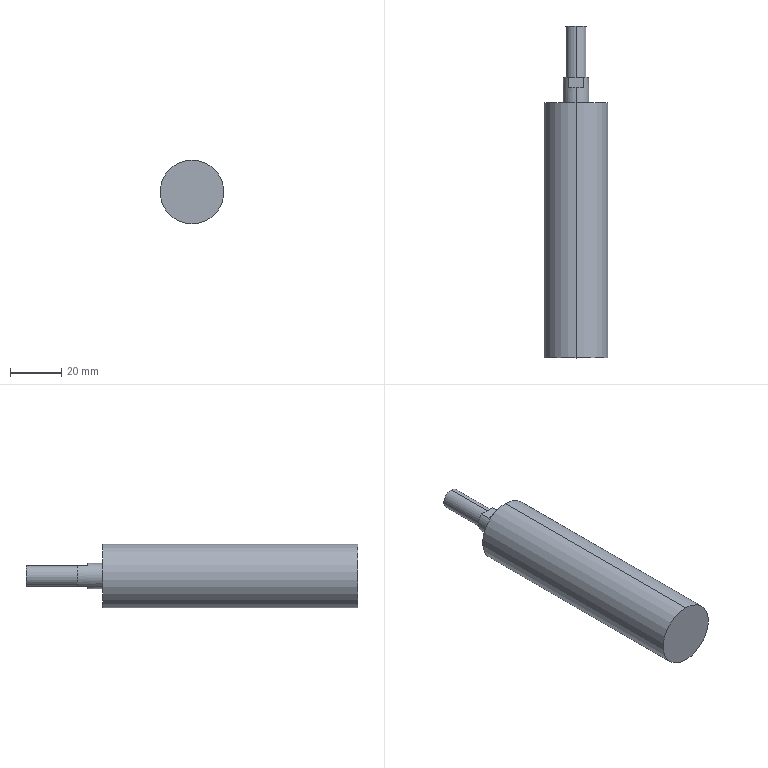Component | SolidWorks | GuideMechanism-1_-StainlessSteelRoller(Vertical)-7 | 1 solid | 15 faces | box 25 x 130 x 25 mm | volume 50845 mm3 | plane 9 | cylinder 6 | commonest cylinder face diameters 8 x2 10 x2 25 x2
build123d program:
from build123d import *

# Parameters (mm, degrees)
SKETCH1_R           = 12.5
BOSS_EXTRUDE1_DEPTH = 50
SKETCH2_R           = 5
BOSS_EXTRUDE2_DEPTH = 10
SKETCH3_R           = 4
BOSS_EXTRUDE3_DEPTH = 20
SKETCH4_W           = 8.872
SKETCH4_H           = 22.159
SKETCH4_W_2         = 4.194
SKETCH4_H_2         = 27.238
CUT_EXTRUDE1_DEPTH  = 4


with BuildPart() as part:
    # Sketch1 → Boss-Extrude1 (new, symmetric)
    with BuildSketch(Plane(origin=(0, 0, 0), x_dir=(0, 0, -1), z_dir=(1, 0, 0))):
        Circle(SKETCH1_R)
    extrude(amount=BOSS_EXTRUDE1_DEPTH, both=True)

    # Sketch2 → Boss-Extrude2 (add)
    with BuildSketch(Plane.ZY.offset(50)):
        with Locations(Location((0, 0, 0), (0, 0, 180))):
            Circle(SKETCH2_R)
    extrude(amount=BOSS_EXTRUDE2_DEPTH)

    # Sketch3 → Boss-Extrude3 (add)
    with BuildSketch(Plane.ZY.offset(60)):
        Circle(SKETCH3_R)
    extrude(amount=BOSS_EXTRUDE3_DEPTH)

    # Sketch4 → Cut-Extrude1 (cut)
    with BuildSketch(Plane.ZY.offset(60)):
        with Locations((8.436, -0.7635)):
            Rectangle(SKETCH4_W, SKETCH4_H)
        with Locations((-6.097, 1.655)):
            Rectangle(SKETCH4_W_2, SKETCH4_H_2)
    extrude(amount=-CUT_EXTRUDE1_DEPTH, mode=Mode.SUBTRACT)


solid = part.part

# Placed as in the assembly
solid = solid.moved(Location((-496.772, -309.766, 1161.5), (0, 0, -90)))
STEP:
#1=COLOUR_RGB('',0.7922,0.8196,0.9333);
#2=FILL_AREA_STYLE_COLOUR('',#1);
#3=FILL_AREA_STYLE('',(#2));
#4=SURFACE_STYLE_FILL_AREA(#3);
#5=SURFACE_SIDE_STYLE('',(#4));
#6=SURFACE_STYLE_USAGE(.BOTH.,#5);
#7=PRESENTATION_STYLE_ASSIGNMENT((#6));
#8=CARTESIAN_POINT('',(-19.558,-9.046,45.571));
#9=VERTEX_POINT('',#8);
#10=CARTESIAN_POINT('',(-19.558,-9.046,45.886));
#11=VERTEX_POINT('',#10);
#12=CARTESIAN_POINT('',(-19.558,-9.046,45.728));
#13=DIRECTION('',(-0.,1.,0.));
#14=DIRECTION('',(0.,0.,-1.));
#15=AXIS2_PLACEMENT_3D('',#12,#13,#14);
#16=CIRCLE('',#15,0.1575);
#17=EDGE_CURVE('',#9,#11,#16,.T.);
#18=ORIENTED_EDGE('',*,*,#17,.F.);
#19=CARTESIAN_POINT('',(-19.558,-9.833,45.571));
#20=VERTEX_POINT('',#19);
#21=CARTESIAN_POINT('',(-19.558,-9.046,45.571));
#22=DIRECTION('',(0.,-1.,-0.));
#23=VECTOR('',#22,39.37);
#24=LINE('',#21,#23);
#25=EDGE_CURVE('',#9,#20,#24,.T.);
#26=ORIENTED_EDGE('',*,*,#25,.T.);
#27=CARTESIAN_POINT('',(-19.558,-9.833,45.886));
#28=VERTEX_POINT('',#27);
#29=CARTESIAN_POINT('',(-19.558,-9.833,45.728));
#30=DIRECTION('',(-0.,1.,0.));
#31=DIRECTION('',(0.,0.,-1.));
#32=AXIS2_PLACEMENT_3D('',#29,#30,#31);
#33=CIRCLE('',#32,0.1575);
#34=EDGE_CURVE('',#20,#28,#33,.T.);
#35=ORIENTED_EDGE('',*,*,#34,.T.);
#36=CARTESIAN_POINT('',(-19.558,-9.046,45.886));
#37=DIRECTION('',(0.,-1.,-0.));
#38=VECTOR('',#37,39.37);
#39=LINE('',#36,#38);
#40=EDGE_CURVE('',#11,#28,#39,.T.);
#41=ORIENTED_EDGE('',*,*,#40,.F.);
#42=EDGE_LOOP('',(#18,#26,#35,#41));
#43=FACE_OUTER_BOUND('',#42,.T.);
#44=CARTESIAN_POINT('',(-19.558,-9.046,45.728));
#45=DIRECTION('',(0.,-1.,-0.));
#46=DIRECTION('',(0.,0.,1.));
#47=AXIS2_PLACEMENT_3D('',#44,#45,#46);
#48=CYLINDRICAL_SURFACE('',#47,0.1575);
#49=ADVANCED_FACE('',(#43),#48,.T.);
#50=CARTESIAN_POINT('',(-19.676,-9.991,45.571));
#51=VERTEX_POINT('',#50);
#52=CARTESIAN_POINT('',(-19.558,-9.991,45.531));
#53=VERTEX_POINT('',#52);
#54=CARTESIAN_POINT('',(-19.558,-9.991,45.728));
#55=DIRECTION('',(0.,-1.,-0.));
#56=DIRECTION('',(0.,0.,1.));
#57=AXIS2_PLACEMENT_3D('',#54,#55,#56);
#58=CIRCLE('',#57,0.1969);
#59=EDGE_CURVE('',#51,#53,#58,.T.);
#60=ORIENTED_EDGE('',*,*,#59,.T.);
#61=CARTESIAN_POINT('',(-19.558,-10.227,45.531));
#62=VERTEX_POINT('',#61);
#63=CARTESIAN_POINT('',(-19.558,-9.833,45.531));
#64=DIRECTION('',(0.,-1.,-0.));
#65=VECTOR('',#64,39.37);
#66=LINE('',#63,#65);
#67=EDGE_CURVE('',#53,#62,#66,.T.);
#68=ORIENTED_EDGE('',*,*,#67,.T.);
#69=CARTESIAN_POINT('',(-19.558,-10.227,45.925));
#70=VERTEX_POINT('',#69);
#71=CARTESIAN_POINT('',(-19.558,-10.227,45.728));
#72=DIRECTION('',(-0.,1.,0.));
#73=DIRECTION('',(0.,0.,1.));
#74=AXIS2_PLACEMENT_3D('',#71,#72,#73);
#75=CIRCLE('',#74,0.1969);
#76=EDGE_CURVE('',#62,#70,#75,.T.);
#77=ORIENTED_EDGE('',*,*,#76,.T.);
#78=CARTESIAN_POINT('',(-19.558,-9.991,45.925));
#79=VERTEX_POINT('',#78);
#80=CARTESIAN_POINT('',(-19.558,-9.833,45.925));
#81=DIRECTION('',(0.,-1.,-0.));
#82=VECTOR('',#81,39.37);
#83=LINE('',#80,#82);
#84=EDGE_CURVE('',#79,#70,#83,.T.);
#85=ORIENTED_EDGE('',*,*,#84,.F.);
#86=CARTESIAN_POINT('',(-19.676,-9.991,45.886));
#87=VERTEX_POINT('',#86);
#88=CARTESIAN_POINT('',(-19.558,-9.991,45.728));
#89=DIRECTION('',(-0.,1.,0.));
#90=DIRECTION('',(0.,0.,-1.));
#91=AXIS2_PLACEMENT_3D('',#88,#89,#90);
#92=CIRCLE('',#91,0.1969);
#93=EDGE_CURVE('',#87,#79,#92,.T.);
#94=ORIENTED_EDGE('',*,*,#93,.F.);
#95=CARTESIAN_POINT('',(-19.676,-9.833,45.886));
#96=VERTEX_POINT('',#95);
#97=CARTESIAN_POINT('',(-19.676,-9.833,45.886));
#98=DIRECTION('',(-0.,1.,0.));
#99=VECTOR('',#98,39.37);
#100=LINE('',#97,#99);
#101=EDGE_CURVE('',#87,#96,#100,.T.);
#102=ORIENTED_EDGE('',*,*,#101,.T.);
#103=CARTESIAN_POINT('',(-19.676,-9.833,45.571));
#104=VERTEX_POINT('',#103);
#105=CARTESIAN_POINT('',(-19.558,-9.833,45.728));
#106=DIRECTION('',(-0.,1.,0.));
#107=DIRECTION('',(0.,0.,-1.));
#108=AXIS2_PLACEMENT_3D('',#105,#106,#107);
#109=CIRCLE('',#108,0.1969);
#110=EDGE_CURVE('',#104,#96,#109,.T.);
#111=ORIENTED_EDGE('',*,*,#110,.F.);
#112=CARTESIAN_POINT('',(-19.676,-9.833,45.571));
#113=DIRECTION('',(0.,-1.,-0.));
#114=VECTOR('',#113,39.37);
#115=LINE('',#112,#114);
#116=EDGE_CURVE('',#104,#51,#115,.T.);
#117=ORIENTED_EDGE('',*,*,#116,.T.);
#118=EDGE_LOOP('',(#60,#68,#77,#85,#94,#102,#111,#117));
#119=FACE_OUTER_BOUND('',#118,.T.);
#120=CARTESIAN_POINT('',(-19.558,-9.833,45.728));
#121=DIRECTION('',(0.,-1.,-0.));
#122=DIRECTION('',(0.,0.,1.));
#123=AXIS2_PLACEMENT_3D('',#120,#121,#122);
#124=CYLINDRICAL_SURFACE('',#123,0.1969);
#125=ADVANCED_FACE('',(#119),#124,.T.);
#126=CARTESIAN_POINT('',(-19.558,-14.164,46.22));
#127=VERTEX_POINT('',#126);
#128=CARTESIAN_POINT('',(-19.558,-14.164,45.236));
#129=VERTEX_POINT('',#128);
#130=CARTESIAN_POINT('',(-19.558,-14.164,45.728));
#131=DIRECTION('',(0.,-1.,-0.));
#132=DIRECTION('',(0.,0.,1.));
#133=AXIS2_PLACEMENT_3D('',#130,#131,#132);
#134=CIRCLE('',#133,0.4921);
#135=EDGE_CURVE('',#127,#129,#134,.T.);
#136=ORIENTED_EDGE('',*,*,#135,.F.);
#137=CARTESIAN_POINT('',(-19.558,-10.227,46.22));
#138=VERTEX_POINT('',#137);
#139=CARTESIAN_POINT('',(-19.558,-14.164,46.22));
#140=DIRECTION('',(-0.,1.,0.));
#141=VECTOR('',#140,39.37);
#142=LINE('',#139,#141);
#143=EDGE_CURVE('',#127,#138,#142,.T.);
#144=ORIENTED_EDGE('',*,*,#143,.T.);
#145=CARTESIAN_POINT('',(-19.558,-10.227,45.236));
#146=VERTEX_POINT('',#145);
#147=CARTESIAN_POINT('',(-19.558,-10.227,45.728));
#148=DIRECTION('',(0.,-1.,-0.));
#149=DIRECTION('',(0.,0.,1.));
#150=AXIS2_PLACEMENT_3D('',#147,#148,#149);
#151=CIRCLE('',#150,0.4921);
#152=EDGE_CURVE('',#138,#146,#151,.T.);
#153=ORIENTED_EDGE('',*,*,#152,.T.);
#154=CARTESIAN_POINT('',(-19.558,-14.164,45.236));
#155=DIRECTION('',(-0.,1.,0.));
#156=VECTOR('',#155,39.37);
#157=LINE('',#154,#156);
#158=EDGE_CURVE('',#129,#146,#157,.T.);
#159=ORIENTED_EDGE('',*,*,#158,.F.);
#160=EDGE_LOOP('',(#136,#144,#153,#159));
#161=FACE_OUTER_BOUND('',#160,.T.);
#162=CARTESIAN_POINT('',(-19.558,-14.164,45.728));
#163=DIRECTION('',(-0.,1.,0.));
#164=DIRECTION('',(0.,0.,-1.));
#165=AXIS2_PLACEMENT_3D('',#162,#163,#164);
#166=CYLINDRICAL_SURFACE('',#165,0.4921);
#167=ADVANCED_FACE('',(#161),#166,.T.);
#168=CARTESIAN_POINT('',(-19.44,-9.833,45.886));
#169=VERTEX_POINT('',#168);
#170=CARTESIAN_POINT('',(-20.159,-9.833,45.886));
#171=DIRECTION('',(-1.,-0.,0.));
#172=VECTOR('',#171,39.37);
#173=LINE('',#170,#172);
#174=EDGE_CURVE('',#169,#28,#173,.T.);
#175=ORIENTED_EDGE('',*,*,#174,.F.);
#176=CARTESIAN_POINT('',(-19.44,-9.833,45.571));
#177=VERTEX_POINT('',#176);
#178=CARTESIAN_POINT('',(-19.558,-9.833,45.728));
#179=DIRECTION('',(-0.,1.,0.));
#180=DIRECTION('',(0.,0.,-1.));
#181=AXIS2_PLACEMENT_3D('',#178,#179,#180);
#182=CIRCLE('',#181,0.1969);
#183=EDGE_CURVE('',#169,#177,#182,.T.);
#184=ORIENTED_EDGE('',*,*,#183,.T.);
#185=CARTESIAN_POINT('',(-19.964,-9.833,45.571));
#186=DIRECTION('',(1.,0.,-0.));
#187=VECTOR('',#186,39.37);
#188=LINE('',#185,#187);
#189=EDGE_CURVE('',#20,#177,#188,.T.);
#190=ORIENTED_EDGE('',*,*,#189,.F.);
#191=CARTESIAN_POINT('',(-19.558,-9.833,45.728));
#192=DIRECTION('',(-0.,1.,0.));
#193=DIRECTION('',(0.,0.,-1.));
#194=AXIS2_PLACEMENT_3D('',#191,#192,#193);
#195=CIRCLE('',#194,0.1575);
#196=EDGE_CURVE('',#28,#20,#195,.T.);
#197=ORIENTED_EDGE('',*,*,#196,.F.);
#198=EDGE_LOOP('',(#175,#184,#190,#197));
#199=FACE_OUTER_BOUND('',#198,.T.);
#200=CARTESIAN_POINT('',(-19.558,-9.833,45.728));
#201=DIRECTION('',(-0.,1.,0.));
#202=DIRECTION('',(0.,0.,-1.));
#203=AXIS2_PLACEMENT_3D('',#200,#201,#202);
#204=PLANE('',#203);
#205=ADVANCED_FACE('',(#199),#204,.T.);
#206=ORIENTED_EDGE('',*,*,#143,.F.);
#207=CARTESIAN_POINT('',(-19.558,-14.164,45.728));
#208=DIRECTION('',(0.,-1.,-0.));
#209=DIRECTION('',(0.,0.,1.));
#210=AXIS2_PLACEMENT_3D('',#207,#208,#209);
#211=CIRCLE('',#210,0.4921);
#212=EDGE_CURVE('',#129,#127,#211,.T.);
#213=ORIENTED_EDGE('',*,*,#212,.F.);
#214=ORIENTED_EDGE('',*,*,#158,.T.);
#215=CARTESIAN_POINT('',(-19.558,-10.227,45.728));
#216=DIRECTION('',(0.,-1.,-0.));
#217=DIRECTION('',(0.,0.,1.));
#218=AXIS2_PLACEMENT_3D('',#215,#216,#217);
#219=CIRCLE('',#218,0.4921);
#220=EDGE_CURVE('',#146,#138,#219,.T.);
#221=ORIENTED_EDGE('',*,*,#220,.T.);
#222=EDGE_LOOP('',(#206,#213,#214,#221));
#223=FACE_OUTER_BOUND('',#222,.T.);
#224=CARTESIAN_POINT('',(-19.558,-14.164,45.728));
#225=DIRECTION('',(-0.,1.,0.));
#226=DIRECTION('',(0.,0.,-1.));
#227=AXIS2_PLACEMENT_3D('',#224,#225,#226);
#228=CYLINDRICAL_SURFACE('',#227,0.4921);
#229=ADVANCED_FACE('',(#223),#228,.T.);
#230=ORIENTED_EDGE('',*,*,#212,.T.);
#231=ORIENTED_EDGE('',*,*,#135,.T.);
#232=EDGE_LOOP('',(#230,#231));
#233=FACE_OUTER_BOUND('',#232,.T.);
#234=CARTESIAN_POINT('',(-19.558,-14.164,45.728));
#235=DIRECTION('',(0.,-1.,-0.));
#236=DIRECTION('',(0.,-0.,1.));
#237=AXIS2_PLACEMENT_3D('',#234,#235,#236);
#238=PLANE('',#237);
#239=ADVANCED_FACE('',(#233),#238,.T.);
#240=CARTESIAN_POINT('',(-19.558,-10.227,45.728));
#241=DIRECTION('',(-0.,1.,0.));
#242=DIRECTION('',(0.,0.,1.));
#243=AXIS2_PLACEMENT_3D('',#240,#241,#242);
#244=CIRCLE('',#243,0.1969);
#245=EDGE_CURVE('',#70,#62,#244,.T.);
#246=ORIENTED_EDGE('',*,*,#245,.F.);
#247=ORIENTED_EDGE('',*,*,#76,.F.);
#248=EDGE_LOOP('',(#246,#247));
#249=FACE_BOUND('',#248,.T.);
#250=ORIENTED_EDGE('',*,*,#220,.F.);
#251=ORIENTED_EDGE('',*,*,#152,.F.);
#252=EDGE_LOOP('',(#250,#251));
#253=FACE_OUTER_BOUND('',#252,.T.);
#254=CARTESIAN_POINT('',(-19.558,-10.227,45.728));
#255=DIRECTION('',(0.,-1.,-0.));
#256=DIRECTION('',(0.,-0.,1.));
#257=AXIS2_PLACEMENT_3D('',#254,#255,#256);
#258=PLANE('',#257);
#259=ADVANCED_FACE('',(#249,#253),#258,.F.);
#260=ORIENTED_EDGE('',*,*,#67,.F.);
#261=CARTESIAN_POINT('',(-19.44,-9.991,45.571));
#262=VERTEX_POINT('',#261);
#263=CARTESIAN_POINT('',(-19.558,-9.991,45.728));
#264=DIRECTION('',(0.,-1.,-0.));
#265=DIRECTION('',(0.,0.,1.));
#266=AXIS2_PLACEMENT_3D('',#263,#264,#265);
#267=CIRCLE('',#266,0.1969);
#268=EDGE_CURVE('',#53,#262,#267,.T.);
#269=ORIENTED_EDGE('',*,*,#268,.T.);
#270=CARTESIAN_POINT('',(-19.44,-9.833,45.571));
#271=DIRECTION('',(-0.,1.,0.));
#272=VECTOR('',#271,39.37);
#273=LINE('',#270,#272);
#274=EDGE_CURVE('',#262,#177,#273,.T.);
#275=ORIENTED_EDGE('',*,*,#274,.T.);
#276=ORIENTED_EDGE('',*,*,#183,.F.);
#277=CARTESIAN_POINT('',(-19.44,-9.991,45.886));
#278=VERTEX_POINT('',#277);
#279=CARTESIAN_POINT('',(-19.44,-9.833,45.886));
#280=DIRECTION('',(0.,-1.,-0.));
#281=VECTOR('',#280,39.37);
#282=LINE('',#279,#281);
#283=EDGE_CURVE('',#169,#278,#282,.T.);
#284=ORIENTED_EDGE('',*,*,#283,.T.);
#285=CARTESIAN_POINT('',(-19.558,-9.991,45.728));
#286=DIRECTION('',(-0.,1.,0.));
#287=DIRECTION('',(0.,0.,-1.));
#288=AXIS2_PLACEMENT_3D('',#285,#286,#287);
#289=CIRCLE('',#288,0.1969);
#290=EDGE_CURVE('',#79,#278,#289,.T.);
#291=ORIENTED_EDGE('',*,*,#290,.F.);
#292=ORIENTED_EDGE('',*,*,#84,.T.);
#293=ORIENTED_EDGE('',*,*,#245,.T.);
#294=EDGE_LOOP('',(#260,#269,#275,#276,#284,#291,#292,#293));
#295=FACE_OUTER_BOUND('',#294,.T.);
#296=CARTESIAN_POINT('',(-19.558,-9.833,45.728));
#297=DIRECTION('',(0.,-1.,-0.));
#298=DIRECTION('',(0.,0.,1.));
#299=AXIS2_PLACEMENT_3D('',#296,#297,#298);
#300=CYLINDRICAL_SURFACE('',#299,0.1969);
#301=ADVANCED_FACE('',(#295),#300,.T.);
#302=CARTESIAN_POINT('',(-20.159,-9.833,45.886));
#303=DIRECTION('',(-1.,-0.,0.));
#304=VECTOR('',#303,39.37);
#305=LINE('',#302,#304);
#306=EDGE_CURVE('',#28,#96,#305,.T.);
#307=ORIENTED_EDGE('',*,*,#306,.F.);
#308=ORIENTED_EDGE('',*,*,#34,.F.);
#309=CARTESIAN_POINT('',(-19.964,-9.833,45.571));
#310=DIRECTION('',(1.,0.,-0.));
#311=VECTOR('',#310,39.37);
#312=LINE('',#309,#311);
#313=EDGE_CURVE('',#104,#20,#312,.T.);
#314=ORIENTED_EDGE('',*,*,#313,.F.);
#315=ORIENTED_EDGE('',*,*,#110,.T.);
#316=EDGE_LOOP('',(#307,#308,#314,#315));
#317=FACE_OUTER_BOUND('',#316,.T.);
#318=CARTESIAN_POINT('',(-19.558,-9.833,45.728));
#319=DIRECTION('',(-0.,1.,0.));
#320=DIRECTION('',(0.,0.,-1.));
#321=AXIS2_PLACEMENT_3D('',#318,#319,#320);
#322=PLANE('',#321);
#323=ADVANCED_FACE('',(#317),#322,.T.);
#324=ORIENTED_EDGE('',*,*,#25,.F.);
#325=CARTESIAN_POINT('',(-19.558,-9.046,45.728));
#326=DIRECTION('',(-0.,1.,0.));
#327=DIRECTION('',(0.,0.,-1.));
#328=AXIS2_PLACEMENT_3D('',#325,#326,#327);
#329=CIRCLE('',#328,0.1575);
#330=EDGE_CURVE('',#11,#9,#329,.T.);
#331=ORIENTED_EDGE('',*,*,#330,.F.);
#332=ORIENTED_EDGE('',*,*,#40,.T.);
#333=ORIENTED_EDGE('',*,*,#196,.T.);
#334=EDGE_LOOP('',(#324,#331,#332,#333));
#335=FACE_OUTER_BOUND('',#334,.T.);
#336=CARTESIAN_POINT('',(-19.558,-9.046,45.728));
#337=DIRECTION('',(0.,-1.,-0.));
#338=DIRECTION('',(0.,0.,1.));
#339=AXIS2_PLACEMENT_3D('',#336,#337,#338);
#340=CYLINDRICAL_SURFACE('',#339,0.1575);
#341=ADVANCED_FACE('',(#335),#340,.T.);
#342=ORIENTED_EDGE('',*,*,#330,.T.);
#343=ORIENTED_EDGE('',*,*,#17,.T.);
#344=EDGE_LOOP('',(#342,#343));
#345=FACE_OUTER_BOUND('',#344,.T.);
#346=CARTESIAN_POINT('',(-19.558,-9.046,45.728));
#347=DIRECTION('',(-0.,1.,0.));
#348=DIRECTION('',(0.,0.,-1.));
#349=AXIS2_PLACEMENT_3D('',#346,#347,#348);
#350=PLANE('',#349);
#351=ADVANCED_FACE('',(#345),#350,.T.);
#352=CARTESIAN_POINT('',(-19.964,-9.991,45.571));
#353=DIRECTION('',(1.,0.,-0.));
#354=VECTOR('',#353,39.37);
#355=LINE('',#352,#354);
#356=EDGE_CURVE('',#51,#262,#355,.T.);
#357=ORIENTED_EDGE('',*,*,#356,.T.);
#358=ORIENTED_EDGE('',*,*,#268,.F.);
#359=ORIENTED_EDGE('',*,*,#59,.F.);
#360=EDGE_LOOP('',(#357,#358,#359));
#361=FACE_OUTER_BOUND('',#360,.T.);
#362=CARTESIAN_POINT('',(-19.558,-9.991,45.728));
#363=DIRECTION('',(0.,-1.,-0.));
#364=DIRECTION('',(0.,-0.,1.));
#365=AXIS2_PLACEMENT_3D('',#362,#363,#364);
#366=PLANE('',#365);
#367=ADVANCED_FACE('',(#361),#366,.F.);
#368=ORIENTED_EDGE('',*,*,#313,.T.);
#369=ORIENTED_EDGE('',*,*,#189,.T.);
#370=ORIENTED_EDGE('',*,*,#274,.F.);
#371=ORIENTED_EDGE('',*,*,#356,.F.);
#372=ORIENTED_EDGE('',*,*,#116,.F.);
#373=EDGE_LOOP('',(#368,#369,#370,#371,#372));
#374=FACE_OUTER_BOUND('',#373,.T.);
#375=CARTESIAN_POINT('',(-19.964,-9.991,45.571));
#376=DIRECTION('',(0.,-0.,1.));
#377=DIRECTION('',(-1.,-0.,0.));
#378=AXIS2_PLACEMENT_3D('',#375,#376,#377);
#379=PLANE('',#378);
#380=ADVANCED_FACE('',(#374),#379,.F.);
#381=ORIENTED_EDGE('',*,*,#93,.T.);
#382=ORIENTED_EDGE('',*,*,#290,.T.);
#383=CARTESIAN_POINT('',(-20.159,-9.991,45.886));
#384=DIRECTION('',(-1.,-0.,0.));
#385=VECTOR('',#384,39.37);
#386=LINE('',#383,#385);
#387=EDGE_CURVE('',#278,#87,#386,.T.);
#388=ORIENTED_EDGE('',*,*,#387,.T.);
#389=EDGE_LOOP('',(#381,#382,#388));
#390=FACE_OUTER_BOUND('',#389,.T.);
#391=CARTESIAN_POINT('',(-19.558,-9.991,45.728));
#392=DIRECTION('',(-0.,1.,0.));
#393=DIRECTION('',(0.,0.,-1.));
#394=AXIS2_PLACEMENT_3D('',#391,#392,#393);
#395=PLANE('',#394);
#396=ADVANCED_FACE('',(#390),#395,.T.);
#397=ORIENTED_EDGE('',*,*,#174,.T.);
#398=ORIENTED_EDGE('',*,*,#306,.T.);
#399=ORIENTED_EDGE('',*,*,#101,.F.);
#400=ORIENTED_EDGE('',*,*,#387,.F.);
#401=ORIENTED_EDGE('',*,*,#283,.F.);
#402=EDGE_LOOP('',(#397,#398,#399,#400,#401));
#403=FACE_OUTER_BOUND('',#402,.T.);
#404=CARTESIAN_POINT('',(-20.159,-9.991,45.886));
#405=DIRECTION('',(-0.,0.,-1.));
#406=DIRECTION('',(1.,0.,-0.));
#407=AXIS2_PLACEMENT_3D('',#404,#405,#406);
#408=PLANE('',#407);
#409=ADVANCED_FACE('',(#403),#408,.F.);
#410=CLOSED_SHELL('',(#49,#125,#167,#205,#229,#239,#259,#301,#323,#341,#351,#367,#380,#396,#409));
#411=MANIFOLD_SOLID_BREP('',#410);
#412=STYLED_ITEM('',(#7),#411);
#413=PRESENTATION_LAYER_ASSIGNMENT('','',(#412));
#414=(LENGTH_UNIT()NAMED_UNIT(*)SI_UNIT($,.METRE.));
#415=LENGTH_MEASURE_WITH_UNIT(LENGTH_MEASURE(0.0254),#414);
#416=DIMENSIONAL_EXPONENTS(1.,0.,0.,0.,0.,0.,0.);
#417=(CONVERSION_BASED_UNIT('',#415)LENGTH_UNIT()NAMED_UNIT(#416));
#418=UNCERTAINTY_MEASURE_WITH_UNIT(LENGTH_MEASURE(0.00001),#417,'','');
#419=(NAMED_UNIT(*)PLANE_ANGLE_UNIT()SI_UNIT($,.RADIAN.));
#420=(NAMED_UNIT(*)SI_UNIT($,.STERADIAN.)SOLID_ANGLE_UNIT());
#421=(GEOMETRIC_REPRESENTATION_CONTEXT(3)GLOBAL_UNCERTAINTY_ASSIGNED_CONTEXT((#418))GLOBAL_UNIT_ASSIGNED_CONTEXT((#417,#419,#420))REPRESENTATION_CONTEXT('',''));
#422=MECHANICAL_DESIGN_GEOMETRIC_PRESENTATION_REPRESENTATION('',(#412),#421);
#423=CARTESIAN_POINT('',(0.,0.,0.));
#424=DIRECTION('',(0.,0.,1.));
#425=DIRECTION('',(1.,0.,0.));
#426=AXIS2_PLACEMENT_3D('',#423,#424,#425);
#427=(LENGTH_UNIT()NAMED_UNIT(*)SI_UNIT($,.METRE.));
#428=LENGTH_MEASURE_WITH_UNIT(LENGTH_MEASURE(0.0254),#427);
#429=DIMENSIONAL_EXPONENTS(1.,0.,0.,0.,0.,0.,0.);
#430=(CONVERSION_BASED_UNIT('',#428)LENGTH_UNIT()NAMED_UNIT(#429));
#431=UNCERTAINTY_MEASURE_WITH_UNIT(LENGTH_MEASURE(0.00001),#430,'','');
#432=(NAMED_UNIT(*)PLANE_ANGLE_UNIT()SI_UNIT($,.RADIAN.));
#433=(NAMED_UNIT(*)SI_UNIT($,.STERADIAN.)SOLID_ANGLE_UNIT());
#434=(GEOMETRIC_REPRESENTATION_CONTEXT(3)GLOBAL_UNCERTAINTY_ASSIGNED_CONTEXT((#431))GLOBAL_UNIT_ASSIGNED_CONTEXT((#430,#432,#433))REPRESENTATION_CONTEXT('',''));
#435=ADVANCED_BREP_SHAPE_REPRESENTATION('',(#411,#426),#434);